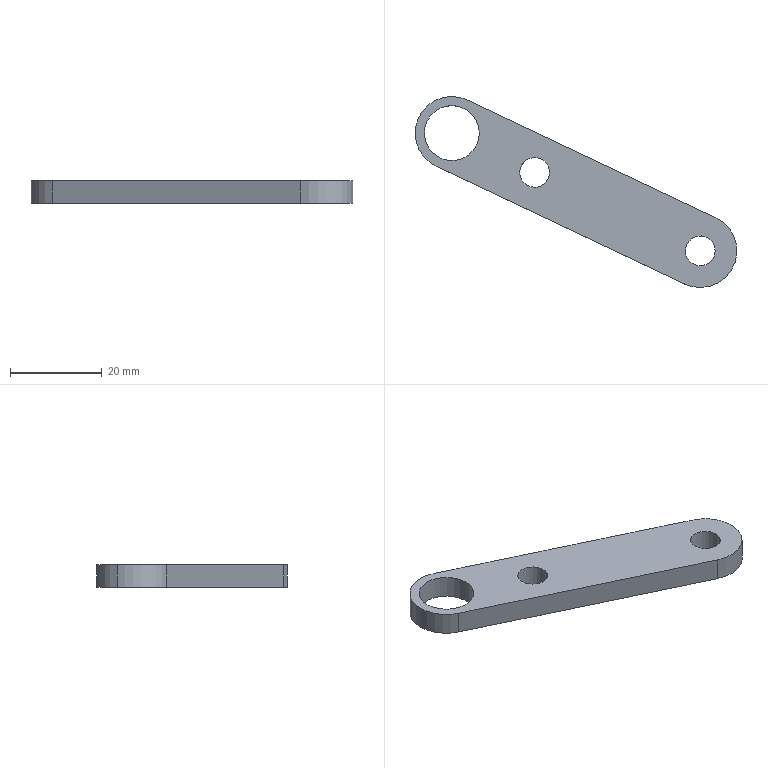Component | SolidWorks | TAR-02-037FixingPlate-1 | 1 solid | 13 faces | box 70.22 x 41.69 x 5 mm | volume 4908 mm3 | cylinder 9 | plane 4 | commonest cylinder face diameters 6.5 x4 16 x3 12 x2
build123d program:
from build123d import *

# Parameters (mm, degrees)
SKETCH1_R           = 3.25
SKETCH1_R_2         = 6
BOSS_EXTRUDE1_DEPTH = 5


with BuildPart() as part:
    # Sketch1 → Boss-Extrude1 (new body)
    with BuildSketch(Plane.XY):
        with BuildLine():
            Line((-30, 8), (30, 8))
            ThreePointArc((30, 8), (38, 0), (30, -8))
            Line((30, -8), (-30, -8))
            ThreePointArc((-30, -8), (-38, 0), (-30, 8))
        make_face()
        with Locations((30, 0)):
            Circle(SKETCH1_R, mode=Mode.SUBTRACT)
        with Locations((-10, 0)):
            Circle(SKETCH1_R, mode=Mode.SUBTRACT)
        with Locations((-30, 0)):
            Circle(SKETCH1_R_2, mode=Mode.SUBTRACT)
    extrude(amount=BOSS_EXTRUDE1_DEPTH)


solid = part.part

# Placed as in the assembly
solid = solid.moved(Location((-18.779, 55.944, -43.165), (0, 0, -25.347)))
STEP:
#1=COLOUR_RGB('',0.7922,0.8196,0.9333);
#2=FILL_AREA_STYLE_COLOUR('',#1);
#3=FILL_AREA_STYLE('',(#2));
#4=SURFACE_STYLE_FILL_AREA(#3);
#5=SURFACE_SIDE_STYLE('',(#4));
#6=SURFACE_STYLE_USAGE(.BOTH.,#5);
#7=PRESENTATION_STYLE_ASSIGNMENT((#6));
#8=CARTESIAN_POINT('',(-2.02,2.809,-1.503));
#9=VERTEX_POINT('',#8);
#10=CARTESIAN_POINT('',(-1.593,2.607,-1.503));
#11=VERTEX_POINT('',#10);
#12=CARTESIAN_POINT('',(-1.807,2.708,-1.503));
#13=DIRECTION('',(0.,0.,1.));
#14=DIRECTION('',(0.9037,-0.4281,0.));
#15=AXIS2_PLACEMENT_3D('',#12,#13,#14);
#16=CIRCLE('',#15,0.2362);
#17=EDGE_CURVE('',#9,#11,#16,.T.);
#18=ORIENTED_EDGE('',*,*,#17,.T.);
#19=CARTESIAN_POINT('',(-1.593,2.607,-1.699));
#20=VERTEX_POINT('',#19);
#21=CARTESIAN_POINT('',(-1.593,2.607,-1.503));
#22=DIRECTION('',(0.,0.,-1.));
#23=VECTOR('',#22,39.37);
#24=LINE('',#21,#23);
#25=EDGE_CURVE('',#11,#20,#24,.T.);
#26=ORIENTED_EDGE('',*,*,#25,.T.);
#27=CARTESIAN_POINT('',(-2.02,2.809,-1.699));
#28=VERTEX_POINT('',#27);
#29=CARTESIAN_POINT('',(-1.807,2.708,-1.699));
#30=DIRECTION('',(0.,0.,1.));
#31=DIRECTION('',(0.9037,-0.4281,0.));
#32=AXIS2_PLACEMENT_3D('',#29,#30,#31);
#33=CIRCLE('',#32,0.2362);
#34=EDGE_CURVE('',#28,#20,#33,.T.);
#35=ORIENTED_EDGE('',*,*,#34,.F.);
#36=CARTESIAN_POINT('',(-2.02,2.809,-1.503));
#37=DIRECTION('',(0.,0.,-1.));
#38=VECTOR('',#37,39.37);
#39=LINE('',#36,#38);
#40=EDGE_CURVE('',#9,#28,#39,.T.);
#41=ORIENTED_EDGE('',*,*,#40,.F.);
#42=EDGE_LOOP('',(#18,#26,#35,#41));
#43=FACE_OUTER_BOUND('',#42,.T.);
#44=CARTESIAN_POINT('',(-1.807,2.708,-1.503));
#45=DIRECTION('',(0.,0.,-1.));
#46=DIRECTION('',(-0.9037,0.4281,0.));
#47=AXIS2_PLACEMENT_3D('',#44,#45,#46);
#48=CYLINDRICAL_SURFACE('',#47,0.2362);
#49=ADVANCED_FACE('',(#43),#48,.F.);
#50=CARTESIAN_POINT('',(-1.211,2.426,-1.503));
#51=VERTEX_POINT('',#50);
#52=CARTESIAN_POINT('',(-0.9795,2.316,-1.503));
#53=VERTEX_POINT('',#52);
#54=CARTESIAN_POINT('',(-1.095,2.371,-1.503));
#55=DIRECTION('',(0.,0.,1.));
#56=DIRECTION('',(0.9037,-0.4281,0.));
#57=AXIS2_PLACEMENT_3D('',#54,#55,#56);
#58=CIRCLE('',#57,0.128);
#59=EDGE_CURVE('',#51,#53,#58,.T.);
#60=ORIENTED_EDGE('',*,*,#59,.T.);
#61=CARTESIAN_POINT('',(-0.9795,2.316,-1.699));
#62=VERTEX_POINT('',#61);
#63=CARTESIAN_POINT('',(-0.9795,2.316,-1.503));
#64=DIRECTION('',(0.,0.,-1.));
#65=VECTOR('',#64,39.37);
#66=LINE('',#63,#65);
#67=EDGE_CURVE('',#53,#62,#66,.T.);
#68=ORIENTED_EDGE('',*,*,#67,.T.);
#69=CARTESIAN_POINT('',(-1.211,2.426,-1.699));
#70=VERTEX_POINT('',#69);
#71=CARTESIAN_POINT('',(-1.095,2.371,-1.699));
#72=DIRECTION('',(0.,0.,1.));
#73=DIRECTION('',(0.9037,-0.4281,0.));
#74=AXIS2_PLACEMENT_3D('',#71,#72,#73);
#75=CIRCLE('',#74,0.128);
#76=EDGE_CURVE('',#70,#62,#75,.T.);
#77=ORIENTED_EDGE('',*,*,#76,.F.);
#78=CARTESIAN_POINT('',(-1.211,2.426,-1.503));
#79=DIRECTION('',(0.,0.,-1.));
#80=VECTOR('',#79,39.37);
#81=LINE('',#78,#80);
#82=EDGE_CURVE('',#51,#70,#81,.T.);
#83=ORIENTED_EDGE('',*,*,#82,.F.);
#84=EDGE_LOOP('',(#60,#68,#77,#83));
#85=FACE_OUTER_BOUND('',#84,.T.);
#86=CARTESIAN_POINT('',(-1.095,2.371,-1.503));
#87=DIRECTION('',(0.,0.,-1.));
#88=DIRECTION('',(-0.9037,0.4281,0.));
#89=AXIS2_PLACEMENT_3D('',#86,#87,#88);
#90=CYLINDRICAL_SURFACE('',#89,0.128);
#91=ADVANCED_FACE('',(#85),#90,.F.);
#92=CARTESIAN_POINT('',(0.2124,1.752,-1.503));
#93=VERTEX_POINT('',#92);
#94=CARTESIAN_POINT('',(0.4437,1.642,-1.503));
#95=VERTEX_POINT('',#94);
#96=CARTESIAN_POINT('',(0.3281,1.697,-1.503));
#97=DIRECTION('',(0.,0.,1.));
#98=DIRECTION('',(0.9037,-0.4281,0.));
#99=AXIS2_PLACEMENT_3D('',#96,#97,#98);
#100=CIRCLE('',#99,0.128);
#101=EDGE_CURVE('',#93,#95,#100,.T.);
#102=ORIENTED_EDGE('',*,*,#101,.T.);
#103=CARTESIAN_POINT('',(0.4437,1.642,-1.699));
#104=VERTEX_POINT('',#103);
#105=CARTESIAN_POINT('',(0.4437,1.642,-1.503));
#106=DIRECTION('',(0.,0.,-1.));
#107=VECTOR('',#106,39.37);
#108=LINE('',#105,#107);
#109=EDGE_CURVE('',#95,#104,#108,.T.);
#110=ORIENTED_EDGE('',*,*,#109,.T.);
#111=CARTESIAN_POINT('',(0.2124,1.752,-1.699));
#112=VERTEX_POINT('',#111);
#113=CARTESIAN_POINT('',(0.3281,1.697,-1.699));
#114=DIRECTION('',(0.,0.,1.));
#115=DIRECTION('',(0.9037,-0.4281,0.));
#116=AXIS2_PLACEMENT_3D('',#113,#114,#115);
#117=CIRCLE('',#116,0.128);
#118=EDGE_CURVE('',#112,#104,#117,.T.);
#119=ORIENTED_EDGE('',*,*,#118,.F.);
#120=CARTESIAN_POINT('',(0.2124,1.752,-1.503));
#121=DIRECTION('',(0.,0.,-1.));
#122=VECTOR('',#121,39.37);
#123=LINE('',#120,#122);
#124=EDGE_CURVE('',#93,#112,#123,.T.);
#125=ORIENTED_EDGE('',*,*,#124,.F.);
#126=EDGE_LOOP('',(#102,#110,#119,#125));
#127=FACE_OUTER_BOUND('',#126,.T.);
#128=CARTESIAN_POINT('',(0.3281,1.697,-1.503));
#129=DIRECTION('',(0.,0.,-1.));
#130=DIRECTION('',(-0.9037,0.4281,0.));
#131=AXIS2_PLACEMENT_3D('',#128,#129,#130);
#132=CYLINDRICAL_SURFACE('',#131,0.128);
#133=ADVANCED_FACE('',(#127),#132,.F.);
#134=CARTESIAN_POINT('',(-2.091,2.843,-1.503));
#135=VERTEX_POINT('',#134);
#136=CARTESIAN_POINT('',(-1.942,2.424,-1.503));
#137=VERTEX_POINT('',#136);
#138=CARTESIAN_POINT('',(-1.807,2.708,-1.503));
#139=DIRECTION('',(0.,0.,1.));
#140=DIRECTION('',(0.9037,-0.4281,0.));
#141=AXIS2_PLACEMENT_3D('',#138,#139,#140);
#142=CIRCLE('',#141,0.315);
#143=EDGE_CURVE('',#135,#137,#142,.T.);
#144=ORIENTED_EDGE('',*,*,#143,.F.);
#145=CARTESIAN_POINT('',(-2.091,2.843,-1.699));
#146=VERTEX_POINT('',#145);
#147=CARTESIAN_POINT('',(-2.091,2.843,-1.503));
#148=DIRECTION('',(0.,0.,-1.));
#149=VECTOR('',#148,39.37);
#150=LINE('',#147,#149);
#151=EDGE_CURVE('',#135,#146,#150,.T.);
#152=ORIENTED_EDGE('',*,*,#151,.T.);
#153=CARTESIAN_POINT('',(-1.942,2.424,-1.699));
#154=VERTEX_POINT('',#153);
#155=CARTESIAN_POINT('',(-1.807,2.708,-1.699));
#156=DIRECTION('',(0.,0.,1.));
#157=DIRECTION('',(0.9037,-0.4281,0.));
#158=AXIS2_PLACEMENT_3D('',#155,#156,#157);
#159=CIRCLE('',#158,0.315);
#160=EDGE_CURVE('',#146,#154,#159,.T.);
#161=ORIENTED_EDGE('',*,*,#160,.T.);
#162=CARTESIAN_POINT('',(-1.942,2.424,-1.503));
#163=DIRECTION('',(0.,0.,-1.));
#164=VECTOR('',#163,39.37);
#165=LINE('',#162,#164);
#166=EDGE_CURVE('',#137,#154,#165,.T.);
#167=ORIENTED_EDGE('',*,*,#166,.F.);
#168=EDGE_LOOP('',(#144,#152,#161,#167));
#169=FACE_OUTER_BOUND('',#168,.T.);
#170=CARTESIAN_POINT('',(-1.807,2.708,-1.503));
#171=DIRECTION('',(0.,0.,-1.));
#172=DIRECTION('',(-0.9037,0.4281,0.));
#173=AXIS2_PLACEMENT_3D('',#170,#171,#172);
#174=CYLINDRICAL_SURFACE('',#173,0.315);
#175=ADVANCED_FACE('',(#169),#174,.T.);
#176=ORIENTED_EDGE('',*,*,#59,.F.);
#177=CARTESIAN_POINT('',(-1.095,2.371,-1.503));
#178=DIRECTION('',(0.,0.,1.));
#179=DIRECTION('',(0.9037,-0.4281,0.));
#180=AXIS2_PLACEMENT_3D('',#177,#178,#179);
#181=CIRCLE('',#180,0.128);
#182=EDGE_CURVE('',#53,#51,#181,.T.);
#183=ORIENTED_EDGE('',*,*,#182,.F.);
#184=EDGE_LOOP('',(#176,#183));
#185=FACE_BOUND('',#184,.T.);
#186=CARTESIAN_POINT('',(-1.672,2.993,-1.503));
#187=VERTEX_POINT('',#186);
#188=CARTESIAN_POINT('',(-1.807,2.708,-1.503));
#189=DIRECTION('',(0.,0.,1.));
#190=DIRECTION('',(0.9037,-0.4281,0.));
#191=AXIS2_PLACEMENT_3D('',#188,#189,#190);
#192=CIRCLE('',#191,0.315);
#193=EDGE_CURVE('',#187,#135,#192,.T.);
#194=ORIENTED_EDGE('',*,*,#193,.T.);
#195=ORIENTED_EDGE('',*,*,#143,.T.);
#196=CARTESIAN_POINT('',(0.1932,1.412,-1.503));
#197=VERTEX_POINT('',#196);
#198=CARTESIAN_POINT('',(-1.942,2.424,-1.503));
#199=DIRECTION('',(0.9037,-0.4281,0.));
#200=VECTOR('',#199,39.37);
#201=LINE('',#198,#200);
#202=EDGE_CURVE('',#137,#197,#201,.T.);
#203=ORIENTED_EDGE('',*,*,#202,.T.);
#204=CARTESIAN_POINT('',(0.4629,1.982,-1.503));
#205=VERTEX_POINT('',#204);
#206=CARTESIAN_POINT('',(0.3281,1.697,-1.503));
#207=DIRECTION('',(0.,0.,1.));
#208=DIRECTION('',(0.9037,-0.4281,0.));
#209=AXIS2_PLACEMENT_3D('',#206,#207,#208);
#210=CIRCLE('',#209,0.315);
#211=EDGE_CURVE('',#197,#205,#210,.T.);
#212=ORIENTED_EDGE('',*,*,#211,.T.);
#213=CARTESIAN_POINT('',(-1.672,2.993,-1.503));
#214=DIRECTION('',(-0.9037,0.4281,0.));
#215=VECTOR('',#214,39.37);
#216=LINE('',#213,#215);
#217=EDGE_CURVE('',#205,#187,#216,.T.);
#218=ORIENTED_EDGE('',*,*,#217,.T.);
#219=EDGE_LOOP('',(#194,#195,#203,#212,#218));
#220=FACE_OUTER_BOUND('',#219,.T.);
#221=ORIENTED_EDGE('',*,*,#101,.F.);
#222=CARTESIAN_POINT('',(0.3281,1.697,-1.503));
#223=DIRECTION('',(0.,0.,1.));
#224=DIRECTION('',(0.9037,-0.4281,0.));
#225=AXIS2_PLACEMENT_3D('',#222,#223,#224);
#226=CIRCLE('',#225,0.128);
#227=EDGE_CURVE('',#95,#93,#226,.T.);
#228=ORIENTED_EDGE('',*,*,#227,.F.);
#229=EDGE_LOOP('',(#221,#228));
#230=FACE_BOUND('',#229,.T.);
#231=ORIENTED_EDGE('',*,*,#17,.F.);
#232=CARTESIAN_POINT('',(-1.807,2.708,-1.503));
#233=DIRECTION('',(0.,0.,1.));
#234=DIRECTION('',(0.9037,-0.4281,0.));
#235=AXIS2_PLACEMENT_3D('',#232,#233,#234);
#236=CIRCLE('',#235,0.2362);
#237=EDGE_CURVE('',#11,#9,#236,.T.);
#238=ORIENTED_EDGE('',*,*,#237,.F.);
#239=EDGE_LOOP('',(#231,#238));
#240=FACE_BOUND('',#239,.T.);
#241=CARTESIAN_POINT('',(-1.807,2.708,-1.503));
#242=DIRECTION('',(0.,0.,1.));
#243=DIRECTION('',(0.9037,-0.4281,0.));
#244=AXIS2_PLACEMENT_3D('',#241,#242,#243);
#245=PLANE('',#244);
#246=ADVANCED_FACE('',(#185,#220,#230,#240),#245,.T.);
#247=CARTESIAN_POINT('',(-1.672,2.993,-1.699));
#248=VERTEX_POINT('',#247);
#249=CARTESIAN_POINT('',(-1.807,2.708,-1.699));
#250=DIRECTION('',(0.,0.,1.));
#251=DIRECTION('',(0.9037,-0.4281,0.));
#252=AXIS2_PLACEMENT_3D('',#249,#250,#251);
#253=CIRCLE('',#252,0.315);
#254=EDGE_CURVE('',#248,#146,#253,.T.);
#255=ORIENTED_EDGE('',*,*,#254,.F.);
#256=CARTESIAN_POINT('',(0.4629,1.982,-1.699));
#257=VERTEX_POINT('',#256);
#258=CARTESIAN_POINT('',(-1.672,2.993,-1.699));
#259=DIRECTION('',(-0.9037,0.4281,0.));
#260=VECTOR('',#259,39.37);
#261=LINE('',#258,#260);
#262=EDGE_CURVE('',#257,#248,#261,.T.);
#263=ORIENTED_EDGE('',*,*,#262,.F.);
#264=CARTESIAN_POINT('',(0.1932,1.412,-1.699));
#265=VERTEX_POINT('',#264);
#266=CARTESIAN_POINT('',(0.3281,1.697,-1.699));
#267=DIRECTION('',(0.,0.,1.));
#268=DIRECTION('',(0.9037,-0.4281,0.));
#269=AXIS2_PLACEMENT_3D('',#266,#267,#268);
#270=CIRCLE('',#269,0.315);
#271=EDGE_CURVE('',#265,#257,#270,.T.);
#272=ORIENTED_EDGE('',*,*,#271,.F.);
#273=CARTESIAN_POINT('',(-1.942,2.424,-1.699));
#274=DIRECTION('',(0.9037,-0.4281,0.));
#275=VECTOR('',#274,39.37);
#276=LINE('',#273,#275);
#277=EDGE_CURVE('',#154,#265,#276,.T.);
#278=ORIENTED_EDGE('',*,*,#277,.F.);
#279=ORIENTED_EDGE('',*,*,#160,.F.);
#280=EDGE_LOOP('',(#255,#263,#272,#278,#279));
#281=FACE_OUTER_BOUND('',#280,.T.);
#282=ORIENTED_EDGE('',*,*,#118,.T.);
#283=CARTESIAN_POINT('',(0.3281,1.697,-1.699));
#284=DIRECTION('',(0.,0.,1.));
#285=DIRECTION('',(0.9037,-0.4281,0.));
#286=AXIS2_PLACEMENT_3D('',#283,#284,#285);
#287=CIRCLE('',#286,0.128);
#288=EDGE_CURVE('',#104,#112,#287,.T.);
#289=ORIENTED_EDGE('',*,*,#288,.T.);
#290=EDGE_LOOP('',(#282,#289));
#291=FACE_BOUND('',#290,.T.);
#292=ORIENTED_EDGE('',*,*,#76,.T.);
#293=CARTESIAN_POINT('',(-1.095,2.371,-1.699));
#294=DIRECTION('',(0.,0.,1.));
#295=DIRECTION('',(0.9037,-0.4281,0.));
#296=AXIS2_PLACEMENT_3D('',#293,#294,#295);
#297=CIRCLE('',#296,0.128);
#298=EDGE_CURVE('',#62,#70,#297,.T.);
#299=ORIENTED_EDGE('',*,*,#298,.T.);
#300=EDGE_LOOP('',(#292,#299));
#301=FACE_BOUND('',#300,.T.);
#302=ORIENTED_EDGE('',*,*,#34,.T.);
#303=CARTESIAN_POINT('',(-1.807,2.708,-1.699));
#304=DIRECTION('',(0.,0.,1.));
#305=DIRECTION('',(0.9037,-0.4281,0.));
#306=AXIS2_PLACEMENT_3D('',#303,#304,#305);
#307=CIRCLE('',#306,0.2362);
#308=EDGE_CURVE('',#20,#28,#307,.T.);
#309=ORIENTED_EDGE('',*,*,#308,.T.);
#310=EDGE_LOOP('',(#302,#309));
#311=FACE_BOUND('',#310,.T.);
#312=CARTESIAN_POINT('',(-1.807,2.708,-1.699));
#313=DIRECTION('',(0.,0.,1.));
#314=DIRECTION('',(0.9037,-0.4281,0.));
#315=AXIS2_PLACEMENT_3D('',#312,#313,#314);
#316=PLANE('',#315);
#317=ADVANCED_FACE('',(#281,#291,#301,#311),#316,.F.);
#318=ORIENTED_EDGE('',*,*,#151,.F.);
#319=ORIENTED_EDGE('',*,*,#193,.F.);
#320=CARTESIAN_POINT('',(-1.672,2.993,-1.503));
#321=DIRECTION('',(0.,0.,-1.));
#322=VECTOR('',#321,39.37);
#323=LINE('',#320,#322);
#324=EDGE_CURVE('',#187,#248,#323,.T.);
#325=ORIENTED_EDGE('',*,*,#324,.T.);
#326=ORIENTED_EDGE('',*,*,#254,.T.);
#327=EDGE_LOOP('',(#318,#319,#325,#326));
#328=FACE_OUTER_BOUND('',#327,.T.);
#329=CARTESIAN_POINT('',(-1.807,2.708,-1.503));
#330=DIRECTION('',(0.,0.,-1.));
#331=DIRECTION('',(-0.9037,0.4281,0.));
#332=AXIS2_PLACEMENT_3D('',#329,#330,#331);
#333=CYLINDRICAL_SURFACE('',#332,0.315);
#334=ADVANCED_FACE('',(#328),#333,.T.);
#335=ORIENTED_EDGE('',*,*,#277,.T.);
#336=CARTESIAN_POINT('',(0.1932,1.412,-1.503));
#337=DIRECTION('',(0.,0.,-1.));
#338=VECTOR('',#337,39.37);
#339=LINE('',#336,#338);
#340=EDGE_CURVE('',#197,#265,#339,.T.);
#341=ORIENTED_EDGE('',*,*,#340,.F.);
#342=ORIENTED_EDGE('',*,*,#202,.F.);
#343=ORIENTED_EDGE('',*,*,#166,.T.);
#344=EDGE_LOOP('',(#335,#341,#342,#343));
#345=FACE_OUTER_BOUND('',#344,.T.);
#346=CARTESIAN_POINT('',(-1.942,2.424,-1.503));
#347=DIRECTION('',(0.4281,0.9037,0.));
#348=DIRECTION('',(0.,0.,1.));
#349=AXIS2_PLACEMENT_3D('',#346,#347,#348);
#350=PLANE('',#349);
#351=ADVANCED_FACE('',(#345),#350,.F.);
#352=ORIENTED_EDGE('',*,*,#271,.T.);
#353=CARTESIAN_POINT('',(0.4629,1.982,-1.503));
#354=DIRECTION('',(0.,0.,-1.));
#355=VECTOR('',#354,39.37);
#356=LINE('',#353,#355);
#357=EDGE_CURVE('',#205,#257,#356,.T.);
#358=ORIENTED_EDGE('',*,*,#357,.F.);
#359=ORIENTED_EDGE('',*,*,#211,.F.);
#360=ORIENTED_EDGE('',*,*,#340,.T.);
#361=EDGE_LOOP('',(#352,#358,#359,#360));
#362=FACE_OUTER_BOUND('',#361,.T.);
#363=CARTESIAN_POINT('',(0.3281,1.697,-1.503));
#364=DIRECTION('',(0.,0.,-1.));
#365=DIRECTION('',(-0.9037,0.4281,0.));
#366=AXIS2_PLACEMENT_3D('',#363,#364,#365);
#367=CYLINDRICAL_SURFACE('',#366,0.315);
#368=ADVANCED_FACE('',(#362),#367,.T.);
#369=ORIENTED_EDGE('',*,*,#262,.T.);
#370=ORIENTED_EDGE('',*,*,#324,.F.);
#371=ORIENTED_EDGE('',*,*,#217,.F.);
#372=ORIENTED_EDGE('',*,*,#357,.T.);
#373=EDGE_LOOP('',(#369,#370,#371,#372));
#374=FACE_OUTER_BOUND('',#373,.T.);
#375=CARTESIAN_POINT('',(-1.672,2.993,-1.503));
#376=DIRECTION('',(-0.4281,-0.9037,0.));
#377=DIRECTION('',(0.,0.,-1.));
#378=AXIS2_PLACEMENT_3D('',#375,#376,#377);
#379=PLANE('',#378);
#380=ADVANCED_FACE('',(#374),#379,.F.);
#381=ORIENTED_EDGE('',*,*,#109,.F.);
#382=ORIENTED_EDGE('',*,*,#227,.T.);
#383=ORIENTED_EDGE('',*,*,#124,.T.);
#384=ORIENTED_EDGE('',*,*,#288,.F.);
#385=EDGE_LOOP('',(#381,#382,#383,#384));
#386=FACE_OUTER_BOUND('',#385,.T.);
#387=CARTESIAN_POINT('',(0.3281,1.697,-1.503));
#388=DIRECTION('',(0.,0.,-1.));
#389=DIRECTION('',(-0.9037,0.4281,0.));
#390=AXIS2_PLACEMENT_3D('',#387,#388,#389);
#391=CYLINDRICAL_SURFACE('',#390,0.128);
#392=ADVANCED_FACE('',(#386),#391,.F.);
#393=ORIENTED_EDGE('',*,*,#67,.F.);
#394=ORIENTED_EDGE('',*,*,#182,.T.);
#395=ORIENTED_EDGE('',*,*,#82,.T.);
#396=ORIENTED_EDGE('',*,*,#298,.F.);
#397=EDGE_LOOP('',(#393,#394,#395,#396));
#398=FACE_OUTER_BOUND('',#397,.T.);
#399=CARTESIAN_POINT('',(-1.095,2.371,-1.503));
#400=DIRECTION('',(0.,0.,-1.));
#401=DIRECTION('',(-0.9037,0.4281,0.));
#402=AXIS2_PLACEMENT_3D('',#399,#400,#401);
#403=CYLINDRICAL_SURFACE('',#402,0.128);
#404=ADVANCED_FACE('',(#398),#403,.F.);
#405=ORIENTED_EDGE('',*,*,#25,.F.);
#406=ORIENTED_EDGE('',*,*,#237,.T.);
#407=ORIENTED_EDGE('',*,*,#40,.T.);
#408=ORIENTED_EDGE('',*,*,#308,.F.);
#409=EDGE_LOOP('',(#405,#406,#407,#408));
#410=FACE_OUTER_BOUND('',#409,.T.);
#411=CARTESIAN_POINT('',(-1.807,2.708,-1.503));
#412=DIRECTION('',(0.,0.,-1.));
#413=DIRECTION('',(-0.9037,0.4281,0.));
#414=AXIS2_PLACEMENT_3D('',#411,#412,#413);
#415=CYLINDRICAL_SURFACE('',#414,0.2362);
#416=ADVANCED_FACE('',(#410),#415,.F.);
#417=CLOSED_SHELL('',(#49,#91,#133,#175,#246,#317,#334,#351,#368,#380,#392,#404,#416));
#418=MANIFOLD_SOLID_BREP('',#417);
#419=STYLED_ITEM('',(#7),#418);
#420=PRESENTATION_LAYER_ASSIGNMENT('','',(#419));
#421=(LENGTH_UNIT()NAMED_UNIT(*)SI_UNIT($,.METRE.));
#422=LENGTH_MEASURE_WITH_UNIT(LENGTH_MEASURE(0.0254),#421);
#423=DIMENSIONAL_EXPONENTS(1.,0.,0.,0.,0.,0.,0.);
#424=(CONVERSION_BASED_UNIT('',#422)LENGTH_UNIT()NAMED_UNIT(#423));
#425=UNCERTAINTY_MEASURE_WITH_UNIT(LENGTH_MEASURE(0.00001),#424,'','');
#426=(NAMED_UNIT(*)PLANE_ANGLE_UNIT()SI_UNIT($,.RADIAN.));
#427=(NAMED_UNIT(*)SI_UNIT($,.STERADIAN.)SOLID_ANGLE_UNIT());
#428=(GEOMETRIC_REPRESENTATION_CONTEXT(3)GLOBAL_UNCERTAINTY_ASSIGNED_CONTEXT((#425))GLOBAL_UNIT_ASSIGNED_CONTEXT((#424,#426,#427))REPRESENTATION_CONTEXT('',''));
#429=MECHANICAL_DESIGN_GEOMETRIC_PRESENTATION_REPRESENTATION('',(#419),#428);
#430=CARTESIAN_POINT('',(0.,0.,0.));
#431=DIRECTION('',(0.,0.,1.));
#432=DIRECTION('',(1.,0.,0.));
#433=AXIS2_PLACEMENT_3D('',#430,#431,#432);
#434=(LENGTH_UNIT()NAMED_UNIT(*)SI_UNIT($,.METRE.));
#435=LENGTH_MEASURE_WITH_UNIT(LENGTH_MEASURE(0.0254),#434);
#436=DIMENSIONAL_EXPONENTS(1.,0.,0.,0.,0.,0.,0.);
#437=(CONVERSION_BASED_UNIT('',#435)LENGTH_UNIT()NAMED_UNIT(#436));
#438=UNCERTAINTY_MEASURE_WITH_UNIT(LENGTH_MEASURE(0.00001),#437,'','');
#439=(NAMED_UNIT(*)PLANE_ANGLE_UNIT()SI_UNIT($,.RADIAN.));
#440=(NAMED_UNIT(*)SI_UNIT($,.STERADIAN.)SOLID_ANGLE_UNIT());
#441=(GEOMETRIC_REPRESENTATION_CONTEXT(3)GLOBAL_UNCERTAINTY_ASSIGNED_CONTEXT((#438))GLOBAL_UNIT_ASSIGNED_CONTEXT((#437,#439,#440))REPRESENTATION_CONTEXT('',''));
#442=ADVANCED_BREP_SHAPE_REPRESENTATION('',(#418,#433),#441);